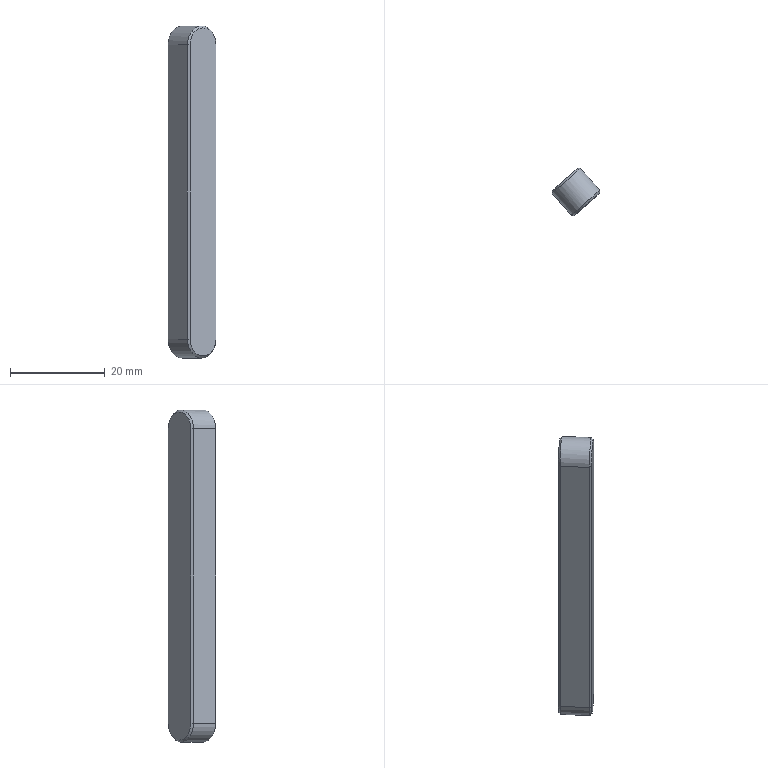Component | SolidWorks | Key8-7-70-1 | 1 solid | 17 faces | box 10.1 x 10.01 x 70 mm | volume 3800 mm3 | plane 8 | cone 6 | cylinder 3 | commonest cylinder face diameters 8 x3
build123d program:
from build123d import *

# Parameters (mm, degrees)
BOSS_EXTRUDE1_DEPTH = 7
CHAMFER1_SIZE2      = 0.4
CHAMFER1_SIZE       = 0.4


with BuildPart() as part:
    # Sketch1 → Boss-Extrude1 (new body)
    with BuildSketch(Plane(origin=(0, 0, 4), x_dir=(1, 0, 0), z_dir=(0, -1, 0))):
        with BuildLine():
            Line((-4, 58), (-4, -4))
            ThreePointArc((-4, -4), (0, -8), (4, -4))
            Line((4, -4), (4, 58))
            ThreePointArc((4, 58), (0, 62), (-4, 58))
        make_face()
    extrude(amount=-BOSS_EXTRUDE1_DEPTH)

    # Chamfer1
    chamfer1_edges = [part.edges().sort_by_distance(p)[0] for p in [
        (0, 7, -4),
        (4, 7, 31),
        (0, 7, 66),
        (4, 0, 31),
        (0, 0, -4),
        (-4, 0, 31),
        (0, 0, 66),
        (-4, 7, 31),
    ]]
    chamfer(chamfer1_edges, length=CHAMFER1_SIZE, length2=CHAMFER1_SIZE2)


solid = part.part

# Placed as in the assembly
solid = solid.moved(Location((-237.022, 13.665, -4.119), (0, 0, -138.66)))
STEP:
#1=COLOUR_RGB('',0.7922,0.8196,0.9333);
#2=FILL_AREA_STYLE_COLOUR('',#1);
#3=FILL_AREA_STYLE('',(#2));
#4=SURFACE_STYLE_FILL_AREA(#3);
#5=SURFACE_SIDE_STYLE('',(#4));
#6=SURFACE_STYLE_USAGE(.BOTH.,#5);
#7=PRESENTATION_STYLE_ASSIGNMENT((#6));
#8=CARTESIAN_POINT('',(-9.332,0.538,-0.3039));
#9=VERTEX_POINT('',#8);
#10=CARTESIAN_POINT('',(-9.438,0.4444,-0.1622));
#11=VERTEX_POINT('',#10);
#12=CARTESIAN_POINT('',(-9.332,0.538,-0.1622));
#13=DIRECTION('',(-0.6605,0.7508,-0.));
#14=DIRECTION('',(0.,0.,-1.));
#15=AXIS2_PLACEMENT_3D('',#12,#13,#14);
#16=CIRCLE('',#15,0.1417);
#17=EDGE_CURVE('',#9,#11,#16,.T.);
#18=ORIENTED_EDGE('',*,*,#17,.F.);
#19=CARTESIAN_POINT('',(-9.321,0.5262,-0.3197));
#20=VERTEX_POINT('',#19);
#21=CARTESIAN_POINT('',(-9.321,0.5262,-0.3197));
#22=DIRECTION('',(0.4671,-0.5309,-0.7071));
#23=VECTOR('',#22,39.37);
#24=LINE('',#21,#23);
#25=EDGE_CURVE('',#9,#20,#24,.T.);
#26=ORIENTED_EDGE('',*,*,#25,.T.);
#27=CARTESIAN_POINT('',(-9.439,0.4221,-0.1622));
#28=VERTEX_POINT('',#27);
#29=CARTESIAN_POINT('',(-9.321,0.5262,-0.1622));
#30=DIRECTION('',(0.6605,-0.7508,0.));
#31=DIRECTION('',(0.,0.,-1.));
#32=AXIS2_PLACEMENT_3D('',#29,#30,#31);
#33=CIRCLE('',#32,0.1575);
#34=EDGE_CURVE('',#28,#20,#33,.T.);
#35=ORIENTED_EDGE('',*,*,#34,.F.);
#36=CARTESIAN_POINT('',(-9.438,0.4444,-0.1622));
#37=DIRECTION('',(-0.06384,-0.998,0.));
#38=VECTOR('',#37,39.37);
#39=LINE('',#36,#38);
#40=EDGE_CURVE('',#11,#28,#39,.T.);
#41=ORIENTED_EDGE('',*,*,#40,.F.);
#42=EDGE_LOOP('',(#18,#26,#35,#41));
#43=FACE_OUTER_BOUND('',#42,.T.);
#44=CARTESIAN_POINT('',(-9.321,0.5262,-0.1622));
#45=DIRECTION('',(0.6605,-0.7508,0.));
#46=DIRECTION('',(0.,0.,-1.));
#47=AXIS2_PLACEMENT_3D('',#44,#45,#46);
#48=CONICAL_SURFACE('',#47,0.1575,0.7854);
#49=ADVANCED_FACE('',(#43),#48,.T.);
#50=CARTESIAN_POINT('',(-9.15,0.3311,2.421));
#51=VERTEX_POINT('',#50);
#52=CARTESIAN_POINT('',(-9.256,0.2374,2.279));
#53=VERTEX_POINT('',#52);
#54=CARTESIAN_POINT('',(-9.15,0.3311,2.279));
#55=DIRECTION('',(0.6605,-0.7508,0.));
#56=DIRECTION('',(0.,0.,-1.));
#57=AXIS2_PLACEMENT_3D('',#54,#55,#56);
#58=CIRCLE('',#57,0.1417);
#59=EDGE_CURVE('',#51,#53,#58,.T.);
#60=ORIENTED_EDGE('',*,*,#59,.F.);
#61=CARTESIAN_POINT('',(-9.16,0.3429,2.436));
#62=VERTEX_POINT('',#61);
#63=CARTESIAN_POINT('',(-9.15,0.3311,2.421));
#64=DIRECTION('',(-0.4671,0.5309,0.7071));
#65=VECTOR('',#64,39.37);
#66=LINE('',#63,#65);
#67=EDGE_CURVE('',#51,#62,#66,.T.);
#68=ORIENTED_EDGE('',*,*,#67,.T.);
#69=CARTESIAN_POINT('',(-9.278,0.2389,2.279));
#70=VERTEX_POINT('',#69);
#71=CARTESIAN_POINT('',(-9.16,0.3429,2.279));
#72=DIRECTION('',(-0.6605,0.7508,-0.));
#73=DIRECTION('',(0.,0.,-1.));
#74=AXIS2_PLACEMENT_3D('',#71,#72,#73);
#75=CIRCLE('',#74,0.1575);
#76=EDGE_CURVE('',#70,#62,#75,.T.);
#77=ORIENTED_EDGE('',*,*,#76,.F.);
#78=CARTESIAN_POINT('',(-9.278,0.2389,2.279));
#79=DIRECTION('',(0.998,-0.06384,0.));
#80=VECTOR('',#79,39.37);
#81=LINE('',#78,#80);
#82=EDGE_CURVE('',#70,#53,#81,.T.);
#83=ORIENTED_EDGE('',*,*,#82,.T.);
#84=EDGE_LOOP('',(#60,#68,#77,#83));
#85=FACE_OUTER_BOUND('',#84,.T.);
#86=CARTESIAN_POINT('',(-9.15,0.3311,2.279));
#87=DIRECTION('',(-0.6605,0.7508,-0.));
#88=DIRECTION('',(0.,0.,1.));
#89=AXIS2_PLACEMENT_3D('',#86,#87,#88);
#90=CONICAL_SURFACE('',#89,0.1417,0.7854);
#91=ADVANCED_FACE('',(#85),#90,.T.);
#92=ORIENTED_EDGE('',*,*,#34,.T.);
#93=CARTESIAN_POINT('',(-9.16,0.3429,-0.3197));
#94=VERTEX_POINT('',#93);
#95=CARTESIAN_POINT('',(-9.332,0.538,-0.3197));
#96=DIRECTION('',(0.6605,-0.7508,0.));
#97=VECTOR('',#96,39.37);
#98=LINE('',#95,#97);
#99=EDGE_CURVE('',#20,#94,#98,.T.);
#100=ORIENTED_EDGE('',*,*,#99,.T.);
#101=CARTESIAN_POINT('',(-9.278,0.2389,-0.1622));
#102=VERTEX_POINT('',#101);
#103=CARTESIAN_POINT('',(-9.16,0.3429,-0.1622));
#104=DIRECTION('',(-0.6605,0.7508,-0.));
#105=DIRECTION('',(0.,-0.,-1.));
#106=AXIS2_PLACEMENT_3D('',#103,#104,#105);
#107=CIRCLE('',#106,0.1575);
#108=EDGE_CURVE('',#94,#102,#107,.T.);
#109=ORIENTED_EDGE('',*,*,#108,.T.);
#110=CARTESIAN_POINT('',(-9.45,0.434,-0.1622));
#111=DIRECTION('',(0.6605,-0.7508,0.));
#112=VECTOR('',#111,39.37);
#113=LINE('',#110,#112);
#114=EDGE_CURVE('',#28,#102,#113,.T.);
#115=ORIENTED_EDGE('',*,*,#114,.F.);
#116=EDGE_LOOP('',(#92,#100,#109,#115));
#117=FACE_OUTER_BOUND('',#116,.T.);
#118=CARTESIAN_POINT('',(-9.332,0.538,-0.1622));
#119=DIRECTION('',(0.6605,-0.7508,0.));
#120=DIRECTION('',(0.,0.,-1.));
#121=AXIS2_PLACEMENT_3D('',#118,#119,#120);
#122=CYLINDRICAL_SURFACE('',#121,0.1575);
#123=ADVANCED_FACE('',(#117),#122,.T.);
#124=CARTESIAN_POINT('',(-9.439,0.4221,2.279));
#125=VERTEX_POINT('',#124);
#126=CARTESIAN_POINT('',(-9.45,0.434,2.279));
#127=DIRECTION('',(0.6605,-0.7508,0.));
#128=VECTOR('',#127,39.37);
#129=LINE('',#126,#128);
#130=EDGE_CURVE('',#125,#70,#129,.T.);
#131=ORIENTED_EDGE('',*,*,#130,.T.);
#132=ORIENTED_EDGE('',*,*,#76,.T.);
#133=CARTESIAN_POINT('',(-9.042,0.4469,2.279));
#134=VERTEX_POINT('',#133);
#135=CARTESIAN_POINT('',(-9.16,0.3429,2.279));
#136=DIRECTION('',(-0.6605,0.7508,-0.));
#137=DIRECTION('',(0.,-0.,-1.));
#138=AXIS2_PLACEMENT_3D('',#135,#136,#137);
#139=CIRCLE('',#138,0.1575);
#140=EDGE_CURVE('',#62,#134,#139,.T.);
#141=ORIENTED_EDGE('',*,*,#140,.T.);
#142=CARTESIAN_POINT('',(-9.203,0.6302,2.279));
#143=VERTEX_POINT('',#142);
#144=CARTESIAN_POINT('',(-9.213,0.642,2.279));
#145=DIRECTION('',(0.6605,-0.7508,0.));
#146=VECTOR('',#145,39.37);
#147=LINE('',#144,#146);
#148=EDGE_CURVE('',#143,#134,#147,.T.);
#149=ORIENTED_EDGE('',*,*,#148,.F.);
#150=CARTESIAN_POINT('',(-9.321,0.5262,2.279));
#151=DIRECTION('',(0.6605,-0.7508,0.));
#152=DIRECTION('',(0.,0.,-1.));
#153=AXIS2_PLACEMENT_3D('',#150,#151,#152);
#154=CIRCLE('',#153,0.1575);
#155=EDGE_CURVE('',#143,#125,#154,.T.);
#156=ORIENTED_EDGE('',*,*,#155,.T.);
#157=EDGE_LOOP('',(#131,#132,#141,#149,#156));
#158=FACE_OUTER_BOUND('',#157,.T.);
#159=CARTESIAN_POINT('',(-9.332,0.538,2.279));
#160=DIRECTION('',(0.6605,-0.7508,0.));
#161=DIRECTION('',(0.,0.,-1.));
#162=AXIS2_PLACEMENT_3D('',#159,#160,#161);
#163=CYLINDRICAL_SURFACE('',#162,0.1575);
#164=ADVANCED_FACE('',(#158),#163,.T.);
#165=ORIENTED_EDGE('',*,*,#148,.T.);
#166=CARTESIAN_POINT('',(-9.042,0.4469,-0.1622));
#167=VERTEX_POINT('',#166);
#168=CARTESIAN_POINT('',(-9.042,0.4469,-0.1622));
#169=DIRECTION('',(0.,-0.,-1.));
#170=VECTOR('',#169,39.37);
#171=LINE('',#168,#170);
#172=EDGE_CURVE('',#134,#167,#171,.T.);
#173=ORIENTED_EDGE('',*,*,#172,.T.);
#174=CARTESIAN_POINT('',(-9.203,0.6302,-0.1622));
#175=VERTEX_POINT('',#174);
#176=CARTESIAN_POINT('',(-9.213,0.642,-0.1622));
#177=DIRECTION('',(0.6605,-0.7508,0.));
#178=VECTOR('',#177,39.37);
#179=LINE('',#176,#178);
#180=EDGE_CURVE('',#175,#167,#179,.T.);
#181=ORIENTED_EDGE('',*,*,#180,.F.);
#182=CARTESIAN_POINT('',(-9.203,0.6302,2.279));
#183=DIRECTION('',(-0.,0.,1.));
#184=VECTOR('',#183,39.37);
#185=LINE('',#182,#184);
#186=EDGE_CURVE('',#175,#143,#185,.T.);
#187=ORIENTED_EDGE('',*,*,#186,.T.);
#188=EDGE_LOOP('',(#165,#173,#181,#187));
#189=FACE_OUTER_BOUND('',#188,.T.);
#190=CARTESIAN_POINT('',(-9.213,0.642,-0.1622));
#191=DIRECTION('',(0.7508,0.6605,0.));
#192=DIRECTION('',(0.,-0.,-1.));
#193=AXIS2_PLACEMENT_3D('',#190,#191,#192);
#194=PLANE('',#193);
#195=ADVANCED_FACE('',(#189),#194,.T.);
#196=ORIENTED_EDGE('',*,*,#99,.F.);
#197=CARTESIAN_POINT('',(-9.321,0.5262,-0.1622));
#198=DIRECTION('',(0.6605,-0.7508,0.));
#199=DIRECTION('',(0.,0.,-1.));
#200=AXIS2_PLACEMENT_3D('',#197,#198,#199);
#201=CIRCLE('',#200,0.1575);
#202=EDGE_CURVE('',#20,#175,#201,.T.);
#203=ORIENTED_EDGE('',*,*,#202,.T.);
#204=ORIENTED_EDGE('',*,*,#180,.T.);
#205=CARTESIAN_POINT('',(-9.16,0.3429,-0.1622));
#206=DIRECTION('',(-0.6605,0.7508,-0.));
#207=DIRECTION('',(0.,0.,-1.));
#208=AXIS2_PLACEMENT_3D('',#205,#206,#207);
#209=CIRCLE('',#208,0.1575);
#210=EDGE_CURVE('',#167,#94,#209,.T.);
#211=ORIENTED_EDGE('',*,*,#210,.T.);
#212=EDGE_LOOP('',(#196,#203,#204,#211));
#213=FACE_OUTER_BOUND('',#212,.T.);
#214=CARTESIAN_POINT('',(-9.332,0.538,-0.1622));
#215=DIRECTION('',(0.6605,-0.7508,0.));
#216=DIRECTION('',(0.,0.,-1.));
#217=AXIS2_PLACEMENT_3D('',#214,#215,#216);
#218=CYLINDRICAL_SURFACE('',#217,0.1575);
#219=ADVANCED_FACE('',(#213),#218,.T.);
#220=ORIENTED_EDGE('',*,*,#114,.T.);
#221=CARTESIAN_POINT('',(-9.278,0.2389,2.279));
#222=DIRECTION('',(-0.,0.,1.));
#223=VECTOR('',#222,39.37);
#224=LINE('',#221,#223);
#225=EDGE_CURVE('',#102,#70,#224,.T.);
#226=ORIENTED_EDGE('',*,*,#225,.T.);
#227=ORIENTED_EDGE('',*,*,#130,.F.);
#228=CARTESIAN_POINT('',(-9.439,0.4221,-0.1622));
#229=DIRECTION('',(0.,-0.,-1.));
#230=VECTOR('',#229,39.37);
#231=LINE('',#228,#230);
#232=EDGE_CURVE('',#125,#28,#231,.T.);
#233=ORIENTED_EDGE('',*,*,#232,.T.);
#234=EDGE_LOOP('',(#220,#226,#227,#233));
#235=FACE_OUTER_BOUND('',#234,.T.);
#236=CARTESIAN_POINT('',(-9.45,0.434,2.279));
#237=DIRECTION('',(-0.7508,-0.6605,-0.));
#238=DIRECTION('',(-0.,0.,1.));
#239=AXIS2_PLACEMENT_3D('',#236,#237,#238);
#240=PLANE('',#239);
#241=ADVANCED_FACE('',(#235),#240,.T.);
#242=CARTESIAN_POINT('',(-9.225,0.6316,-0.1622));
#243=VERTEX_POINT('',#242);
#244=CARTESIAN_POINT('',(-9.332,0.538,-0.1622));
#245=DIRECTION('',(-0.6605,0.7508,-0.));
#246=DIRECTION('',(0.,-0.,-1.));
#247=AXIS2_PLACEMENT_3D('',#244,#245,#246);
#248=CIRCLE('',#247,0.1417);
#249=EDGE_CURVE('',#243,#9,#248,.T.);
#250=ORIENTED_EDGE('',*,*,#249,.T.);
#251=ORIENTED_EDGE('',*,*,#17,.T.);
#252=CARTESIAN_POINT('',(-9.438,0.4444,2.279));
#253=VERTEX_POINT('',#252);
#254=CARTESIAN_POINT('',(-9.438,0.4444,2.279));
#255=DIRECTION('',(-0.,0.,1.));
#256=VECTOR('',#255,39.37);
#257=LINE('',#254,#256);
#258=EDGE_CURVE('',#11,#253,#257,.T.);
#259=ORIENTED_EDGE('',*,*,#258,.T.);
#260=CARTESIAN_POINT('',(-9.225,0.6316,2.279));
#261=VERTEX_POINT('',#260);
#262=CARTESIAN_POINT('',(-9.332,0.538,2.279));
#263=DIRECTION('',(-0.6605,0.7508,-0.));
#264=DIRECTION('',(0.,0.,-1.));
#265=AXIS2_PLACEMENT_3D('',#262,#263,#264);
#266=CIRCLE('',#265,0.1417);
#267=EDGE_CURVE('',#253,#261,#266,.T.);
#268=ORIENTED_EDGE('',*,*,#267,.T.);
#269=CARTESIAN_POINT('',(-9.225,0.6316,-0.1622));
#270=DIRECTION('',(0.,-0.,-1.));
#271=VECTOR('',#270,39.37);
#272=LINE('',#269,#271);
#273=EDGE_CURVE('',#261,#243,#272,.T.);
#274=ORIENTED_EDGE('',*,*,#273,.T.);
#275=EDGE_LOOP('',(#250,#251,#259,#268,#274));
#276=FACE_OUTER_BOUND('',#275,.T.);
#277=CARTESIAN_POINT('',(-9.332,0.538,2.279));
#278=DIRECTION('',(0.6605,-0.7508,0.));
#279=DIRECTION('',(0.,-0.,-1.));
#280=AXIS2_PLACEMENT_3D('',#277,#278,#279);
#281=PLANE('',#280);
#282=ADVANCED_FACE('',(#276),#281,.F.);
#283=CARTESIAN_POINT('',(-9.256,0.2374,-0.1622));
#284=VERTEX_POINT('',#283);
#285=CARTESIAN_POINT('',(-9.043,0.4247,-0.1622));
#286=VERTEX_POINT('',#285);
#287=CARTESIAN_POINT('',(-9.15,0.3311,-0.1622));
#288=DIRECTION('',(0.6605,-0.7508,0.));
#289=DIRECTION('',(0.,0.,-1.));
#290=AXIS2_PLACEMENT_3D('',#287,#288,#289);
#291=CIRCLE('',#290,0.1417);
#292=EDGE_CURVE('',#284,#286,#291,.T.);
#293=ORIENTED_EDGE('',*,*,#292,.T.);
#294=CARTESIAN_POINT('',(-9.043,0.4247,2.279));
#295=VERTEX_POINT('',#294);
#296=CARTESIAN_POINT('',(-9.043,0.4247,2.279));
#297=DIRECTION('',(-0.,0.,1.));
#298=VECTOR('',#297,39.37);
#299=LINE('',#296,#298);
#300=EDGE_CURVE('',#286,#295,#299,.T.);
#301=ORIENTED_EDGE('',*,*,#300,.T.);
#302=CARTESIAN_POINT('',(-9.15,0.3311,2.279));
#303=DIRECTION('',(0.6605,-0.7508,0.));
#304=DIRECTION('',(0.,0.,-1.));
#305=AXIS2_PLACEMENT_3D('',#302,#303,#304);
#306=CIRCLE('',#305,0.1417);
#307=EDGE_CURVE('',#295,#51,#306,.T.);
#308=ORIENTED_EDGE('',*,*,#307,.T.);
#309=ORIENTED_EDGE('',*,*,#59,.T.);
#310=CARTESIAN_POINT('',(-9.256,0.2374,2.279));
#311=DIRECTION('',(0.,-0.,-1.));
#312=VECTOR('',#311,39.37);
#313=LINE('',#310,#312);
#314=EDGE_CURVE('',#53,#284,#313,.T.);
#315=ORIENTED_EDGE('',*,*,#314,.T.);
#316=EDGE_LOOP('',(#293,#301,#308,#309,#315));
#317=FACE_OUTER_BOUND('',#316,.T.);
#318=CARTESIAN_POINT('',(-9.15,0.3311,2.279));
#319=DIRECTION('',(0.6605,-0.7508,0.));
#320=DIRECTION('',(0.,-0.,-1.));
#321=AXIS2_PLACEMENT_3D('',#318,#319,#320);
#322=PLANE('',#321);
#323=ADVANCED_FACE('',(#317),#322,.T.);
#324=ORIENTED_EDGE('',*,*,#82,.F.);
#325=ORIENTED_EDGE('',*,*,#225,.F.);
#326=CARTESIAN_POINT('',(-9.256,0.2374,-0.1622));
#327=DIRECTION('',(-0.998,0.06384,-0.));
#328=VECTOR('',#327,39.37);
#329=LINE('',#326,#328);
#330=EDGE_CURVE('',#284,#102,#329,.T.);
#331=ORIENTED_EDGE('',*,*,#330,.F.);
#332=ORIENTED_EDGE('',*,*,#314,.F.);
#333=EDGE_LOOP('',(#324,#325,#331,#332));
#334=FACE_OUTER_BOUND('',#333,.T.);
#335=CARTESIAN_POINT('',(-9.256,0.2374,2.279));
#336=DIRECTION('',(0.06384,0.998,-0.));
#337=DIRECTION('',(0.,-0.,-1.));
#338=AXIS2_PLACEMENT_3D('',#335,#336,#337);
#339=PLANE('',#338);
#340=ADVANCED_FACE('',(#334),#339,.F.);
#341=ORIENTED_EDGE('',*,*,#330,.T.);
#342=ORIENTED_EDGE('',*,*,#108,.F.);
#343=ORIENTED_EDGE('',*,*,#210,.F.);
#344=CARTESIAN_POINT('',(-9.043,0.4247,-0.1622));
#345=DIRECTION('',(0.06384,0.998,-0.));
#346=VECTOR('',#345,39.37);
#347=LINE('',#344,#346);
#348=EDGE_CURVE('',#286,#167,#347,.T.);
#349=ORIENTED_EDGE('',*,*,#348,.F.);
#350=ORIENTED_EDGE('',*,*,#292,.F.);
#351=EDGE_LOOP('',(#341,#342,#343,#349,#350));
#352=FACE_OUTER_BOUND('',#351,.T.);
#353=CARTESIAN_POINT('',(-9.15,0.3311,-0.1622));
#354=DIRECTION('',(-0.6605,0.7508,-0.));
#355=DIRECTION('',(0.,0.,1.));
#356=AXIS2_PLACEMENT_3D('',#353,#354,#355);
#357=CONICAL_SURFACE('',#356,0.1417,0.7854);
#358=ADVANCED_FACE('',(#352),#357,.T.);
#359=ORIENTED_EDGE('',*,*,#67,.F.);
#360=ORIENTED_EDGE('',*,*,#307,.F.);
#361=CARTESIAN_POINT('',(-9.042,0.4469,2.279));
#362=DIRECTION('',(-0.06384,-0.998,0.));
#363=VECTOR('',#362,39.37);
#364=LINE('',#361,#363);
#365=EDGE_CURVE('',#134,#295,#364,.T.);
#366=ORIENTED_EDGE('',*,*,#365,.F.);
#367=ORIENTED_EDGE('',*,*,#140,.F.);
#368=EDGE_LOOP('',(#359,#360,#366,#367));
#369=FACE_OUTER_BOUND('',#368,.T.);
#370=CARTESIAN_POINT('',(-9.15,0.3311,2.279));
#371=DIRECTION('',(-0.6605,0.7508,-0.));
#372=DIRECTION('',(0.,0.,1.));
#373=AXIS2_PLACEMENT_3D('',#370,#371,#372);
#374=CONICAL_SURFACE('',#373,0.1417,0.7854);
#375=ADVANCED_FACE('',(#369),#374,.T.);
#376=ORIENTED_EDGE('',*,*,#348,.T.);
#377=ORIENTED_EDGE('',*,*,#172,.F.);
#378=ORIENTED_EDGE('',*,*,#365,.T.);
#379=ORIENTED_EDGE('',*,*,#300,.F.);
#380=EDGE_LOOP('',(#376,#377,#378,#379));
#381=FACE_OUTER_BOUND('',#380,.T.);
#382=CARTESIAN_POINT('',(-9.043,0.4247,2.279));
#383=DIRECTION('',(-0.998,0.06384,-0.));
#384=DIRECTION('',(-0.,0.,1.));
#385=AXIS2_PLACEMENT_3D('',#382,#383,#384);
#386=PLANE('',#385);
#387=ADVANCED_FACE('',(#381),#386,.F.);
#388=CARTESIAN_POINT('',(-9.225,0.6316,-0.1622));
#389=DIRECTION('',(0.998,-0.06384,0.));
#390=VECTOR('',#389,39.37);
#391=LINE('',#388,#390);
#392=EDGE_CURVE('',#243,#175,#391,.T.);
#393=ORIENTED_EDGE('',*,*,#392,.F.);
#394=ORIENTED_EDGE('',*,*,#273,.F.);
#395=CARTESIAN_POINT('',(-9.203,0.6302,2.279));
#396=DIRECTION('',(-0.998,0.06384,-0.));
#397=VECTOR('',#396,39.37);
#398=LINE('',#395,#397);
#399=EDGE_CURVE('',#143,#261,#398,.T.);
#400=ORIENTED_EDGE('',*,*,#399,.F.);
#401=ORIENTED_EDGE('',*,*,#186,.F.);
#402=EDGE_LOOP('',(#393,#394,#400,#401));
#403=FACE_OUTER_BOUND('',#402,.T.);
#404=CARTESIAN_POINT('',(-9.203,0.6302,-0.1622));
#405=DIRECTION('',(0.06384,0.998,-0.));
#406=DIRECTION('',(0.,-0.,-1.));
#407=AXIS2_PLACEMENT_3D('',#404,#405,#406);
#408=PLANE('',#407);
#409=ADVANCED_FACE('',(#403),#408,.T.);
#410=ORIENTED_EDGE('',*,*,#399,.T.);
#411=ORIENTED_EDGE('',*,*,#267,.F.);
#412=CARTESIAN_POINT('',(-9.439,0.4221,2.279));
#413=DIRECTION('',(0.06384,0.998,-0.));
#414=VECTOR('',#413,39.37);
#415=LINE('',#412,#414);
#416=EDGE_CURVE('',#125,#253,#415,.T.);
#417=ORIENTED_EDGE('',*,*,#416,.F.);
#418=ORIENTED_EDGE('',*,*,#155,.F.);
#419=EDGE_LOOP('',(#410,#411,#417,#418));
#420=FACE_OUTER_BOUND('',#419,.T.);
#421=CARTESIAN_POINT('',(-9.321,0.5262,2.279));
#422=DIRECTION('',(0.6605,-0.7508,0.));
#423=DIRECTION('',(0.,0.,-1.));
#424=AXIS2_PLACEMENT_3D('',#421,#422,#423);
#425=CONICAL_SURFACE('',#424,0.1575,0.7854);
#426=ADVANCED_FACE('',(#420),#425,.T.);
#427=ORIENTED_EDGE('',*,*,#25,.F.);
#428=ORIENTED_EDGE('',*,*,#249,.F.);
#429=ORIENTED_EDGE('',*,*,#392,.T.);
#430=ORIENTED_EDGE('',*,*,#202,.F.);
#431=EDGE_LOOP('',(#427,#428,#429,#430));
#432=FACE_OUTER_BOUND('',#431,.T.);
#433=CARTESIAN_POINT('',(-9.321,0.5262,-0.1622));
#434=DIRECTION('',(0.6605,-0.7508,0.));
#435=DIRECTION('',(0.,0.,-1.));
#436=AXIS2_PLACEMENT_3D('',#433,#434,#435);
#437=CONICAL_SURFACE('',#436,0.1575,0.7854);
#438=ADVANCED_FACE('',(#432),#437,.T.);
#439=ORIENTED_EDGE('',*,*,#416,.T.);
#440=ORIENTED_EDGE('',*,*,#258,.F.);
#441=ORIENTED_EDGE('',*,*,#40,.T.);
#442=ORIENTED_EDGE('',*,*,#232,.F.);
#443=EDGE_LOOP('',(#439,#440,#441,#442));
#444=FACE_OUTER_BOUND('',#443,.T.);
#445=CARTESIAN_POINT('',(-9.439,0.4221,2.279));
#446=DIRECTION('',(-0.998,0.06384,-0.));
#447=DIRECTION('',(-0.,0.,1.));
#448=AXIS2_PLACEMENT_3D('',#445,#446,#447);
#449=PLANE('',#448);
#450=ADVANCED_FACE('',(#444),#449,.T.);
#451=CLOSED_SHELL('',(#49,#91,#123,#164,#195,#219,#241,#282,#323,#340,#358,#375,#387,#409,#426,#438,#450));
#452=MANIFOLD_SOLID_BREP('',#451);
#453=STYLED_ITEM('',(#7),#452);
#454=(LENGTH_UNIT()NAMED_UNIT(*)SI_UNIT($,.METRE.));
#455=LENGTH_MEASURE_WITH_UNIT(LENGTH_MEASURE(0.0254),#454);
#456=DIMENSIONAL_EXPONENTS(1.,0.,0.,0.,0.,0.,0.);
#457=(CONVERSION_BASED_UNIT('',#455)LENGTH_UNIT()NAMED_UNIT(#456));
#458=UNCERTAINTY_MEASURE_WITH_UNIT(LENGTH_MEASURE(0.00001),#457,'','');
#459=(NAMED_UNIT(*)PLANE_ANGLE_UNIT()SI_UNIT($,.RADIAN.));
#460=(NAMED_UNIT(*)SI_UNIT($,.STERADIAN.)SOLID_ANGLE_UNIT());
#461=(GEOMETRIC_REPRESENTATION_CONTEXT(3)GLOBAL_UNCERTAINTY_ASSIGNED_CONTEXT((#458))GLOBAL_UNIT_ASSIGNED_CONTEXT((#457,#459,#460))REPRESENTATION_CONTEXT('',''));
#462=MECHANICAL_DESIGN_GEOMETRIC_PRESENTATION_REPRESENTATION('',(#453),#461);
#463=PRESENTATION_LAYER_ASSIGNMENT('','',(#453));
#464=CARTESIAN_POINT('',(0.,0.,0.));
#465=DIRECTION('',(0.,0.,1.));
#466=DIRECTION('',(1.,0.,0.));
#467=AXIS2_PLACEMENT_3D('',#464,#465,#466);
#468=(LENGTH_UNIT()NAMED_UNIT(*)SI_UNIT($,.METRE.));
#469=LENGTH_MEASURE_WITH_UNIT(LENGTH_MEASURE(0.0254),#468);
#470=DIMENSIONAL_EXPONENTS(1.,0.,0.,0.,0.,0.,0.);
#471=(CONVERSION_BASED_UNIT('',#469)LENGTH_UNIT()NAMED_UNIT(#470));
#472=UNCERTAINTY_MEASURE_WITH_UNIT(LENGTH_MEASURE(0.00001),#471,'','');
#473=(NAMED_UNIT(*)PLANE_ANGLE_UNIT()SI_UNIT($,.RADIAN.));
#474=(NAMED_UNIT(*)SI_UNIT($,.STERADIAN.)SOLID_ANGLE_UNIT());
#475=(GEOMETRIC_REPRESENTATION_CONTEXT(3)GLOBAL_UNCERTAINTY_ASSIGNED_CONTEXT((#472))GLOBAL_UNIT_ASSIGNED_CONTEXT((#471,#473,#474))REPRESENTATION_CONTEXT('',''));
#476=ADVANCED_BREP_SHAPE_REPRESENTATION('',(#452,#467),#475);